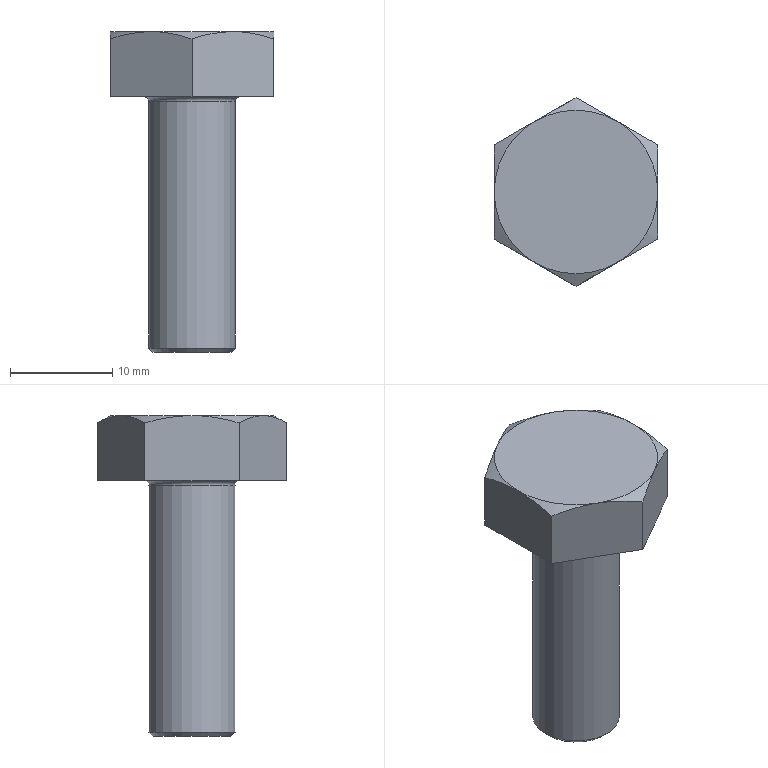Component | NX | GB-T5781-2000_M10X25_3 | 1 solid | 18 faces | volume 2832 mm3 | plane 9 | cone 7 | cylinder 1 | torus 1 | commonest cylinder face diameters 8.5 x1